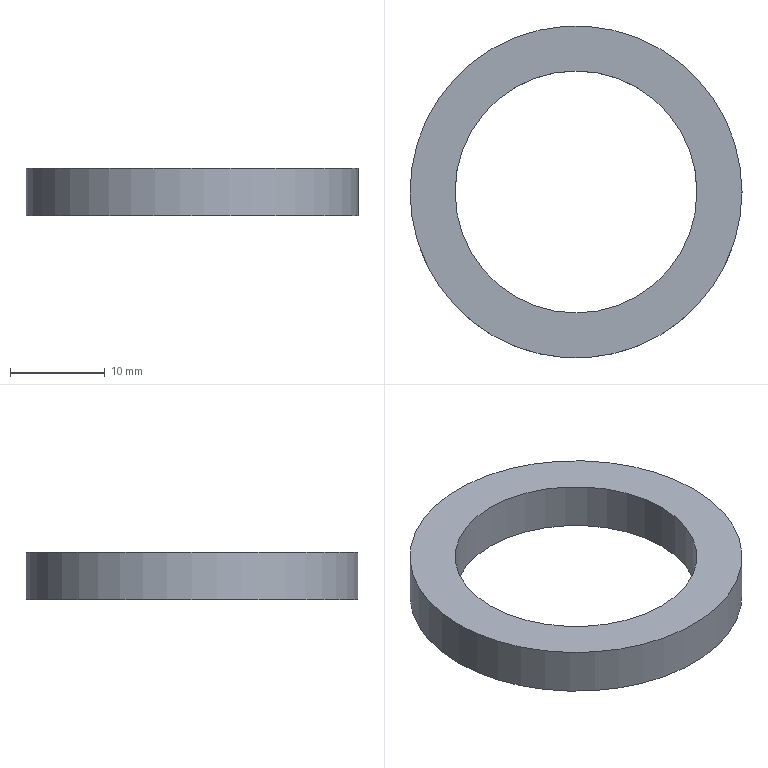Component | NX | SHAFT_SLEEVE_1 | 1 solid | 4 faces | box 35 x 35 x 5 mm | volume 2257 mm3 | cylinder 2 | plane 2 | commonest cylinder face diameters 35 x1 25.5 x1
STEP:
#1=CARTESIAN_POINT('',(0.,0.,0.));
#2=DIRECTION('',(0.,0.,1.));
#3=DIRECTION('',(1.,0.,0.));
#4=AXIS2_PLACEMENT_3D('',#1,#2,#3);
#5=CARTESIAN_POINT('',(-406.675,308.181,-720.));
#6=VERTEX_POINT('',#5);
#7=CARTESIAN_POINT('',(-424.175,308.181,-720.));
#8=DIRECTION('',(0.,0.,1.));
#9=DIRECTION('',(1.,0.,0.));
#10=AXIS2_PLACEMENT_3D('',#7,#8,#9);
#11=CIRCLE('',#10,17.5);
#12=CARTESIAN_POINT('',(-424.175,308.181,-720.));
#13=DIRECTION('',(0.,0.,-1.));
#14=DIRECTION('',(-1.,0.,0.));
#15=AXIS2_PLACEMENT_3D('',#12,#13,#14);
#16=CYLINDRICAL_SURFACE('',#15,17.5);
#17=CARTESIAN_POINT('',(9.425,0.));
#18=DIRECTION('',(-1.,0.));
#19=VECTOR('',#18,1.);
#20=LINE('',#17,#19);
#21=(GEOMETRIC_REPRESENTATION_CONTEXT(2)PARAMETRIC_REPRESENTATION_CONTEXT()REPRESENTATION_CONTEXT('',''));
#22=DEFINITIONAL_REPRESENTATION('',(#20),#21);
#23=PCURVE('',#16,#22);
#24=CARTESIAN_POINT('',(-424.175,308.181,-720.));
#25=DIRECTION('',(0.,0.,1.));
#26=DIRECTION('',(1.,0.,0.));
#27=AXIS2_PLACEMENT_3D('',#24,#25,#26);
#28=PLANE('',#27);
#29=CARTESIAN_POINT('',(0.,0.));
#30=DIRECTION('',(1.,0.));
#31=AXIS2_PLACEMENT_2D('',#29,#30);
#32=CIRCLE('',#31,17.5);
#33=(GEOMETRIC_REPRESENTATION_CONTEXT(2)PARAMETRIC_REPRESENTATION_CONTEXT()REPRESENTATION_CONTEXT('',''));
#34=DEFINITIONAL_REPRESENTATION('',(#32),#33);
#35=PCURVE('',#28,#34);
#36=SURFACE_CURVE('',#11,(#23,#35),.PCURVE_S1.);
#37=EDGE_CURVE('',#6,#6,#36,.T.);
#38=ORIENTED_EDGE('',*,*,#37,.F.);
#39=CARTESIAN_POINT('',(-406.675,308.181,-725.));
#40=VERTEX_POINT('',#39);
#41=CARTESIAN_POINT('',(-406.675,308.181,-720.));
#42=CARTESIAN_POINT('',(-406.675,308.181,-725.));
#43=B_SPLINE_CURVE_WITH_KNOTS('',1,(#41,#42),.UNSPECIFIED.,.F.,.F.,(2,2),(0.,5.),.PIECEWISE_BEZIER_KNOTS.);
#44=CARTESIAN_POINT('',(9.425,0.));
#45=DIRECTION('',(0.,1.));
#46=VECTOR('',#45,1.);
#47=LINE('',#44,#46);
#48=(GEOMETRIC_REPRESENTATION_CONTEXT(2)PARAMETRIC_REPRESENTATION_CONTEXT()REPRESENTATION_CONTEXT('',''));
#49=DEFINITIONAL_REPRESENTATION('',(#47),#48);
#50=PCURVE('',#16,#49);
#51=CARTESIAN_POINT('',(3.142,0.));
#52=DIRECTION('',(0.,1.));
#53=VECTOR('',#52,1.);
#54=LINE('',#51,#53);
#55=(GEOMETRIC_REPRESENTATION_CONTEXT(2)PARAMETRIC_REPRESENTATION_CONTEXT()REPRESENTATION_CONTEXT('',''));
#56=DEFINITIONAL_REPRESENTATION('',(#54),#55);
#57=PCURVE('',#16,#56);
#58=SEAM_CURVE('',#43,(#50,#57),.PCURVE_S1.);
#59=EDGE_CURVE('',#6,#40,#58,.T.);
#60=ORIENTED_EDGE('',*,*,#59,.T.);
#61=CARTESIAN_POINT('',(-424.175,308.181,-725.));
#62=DIRECTION('',(0.,0.,1.));
#63=DIRECTION('',(1.,0.,0.));
#64=AXIS2_PLACEMENT_3D('',#61,#62,#63);
#65=CIRCLE('',#64,17.5);
#66=CARTESIAN_POINT('',(9.425,5.));
#67=DIRECTION('',(-1.,0.));
#68=VECTOR('',#67,1.);
#69=LINE('',#66,#68);
#70=(GEOMETRIC_REPRESENTATION_CONTEXT(2)PARAMETRIC_REPRESENTATION_CONTEXT()REPRESENTATION_CONTEXT('',''));
#71=DEFINITIONAL_REPRESENTATION('',(#69),#70);
#72=PCURVE('',#16,#71);
#73=CARTESIAN_POINT('',(-424.175,308.181,-725.));
#74=DIRECTION('',(0.,0.,1.));
#75=DIRECTION('',(1.,0.,0.));
#76=AXIS2_PLACEMENT_3D('',#73,#74,#75);
#77=PLANE('',#76);
#78=CARTESIAN_POINT('',(0.,0.));
#79=DIRECTION('',(1.,0.));
#80=AXIS2_PLACEMENT_2D('',#78,#79);
#81=CIRCLE('',#80,17.5);
#82=(GEOMETRIC_REPRESENTATION_CONTEXT(2)PARAMETRIC_REPRESENTATION_CONTEXT()REPRESENTATION_CONTEXT('',''));
#83=DEFINITIONAL_REPRESENTATION('',(#81),#82);
#84=PCURVE('',#77,#83);
#85=SURFACE_CURVE('',#65,(#72,#84),.PCURVE_S1.);
#86=EDGE_CURVE('',#40,#40,#85,.T.);
#87=ORIENTED_EDGE('',*,*,#86,.T.);
#88=ORIENTED_EDGE('',*,*,#59,.F.);
#89=EDGE_LOOP('',(#38,#60,#87,#88));
#90=FACE_BOUND('',#89,.T.);
#91=ADVANCED_FACE('',(#90),#16,.T.);
#92=CARTESIAN_POINT('',(-411.425,308.181,-720.));
#93=VERTEX_POINT('',#92);
#94=CARTESIAN_POINT('',(-424.175,308.181,-720.));
#95=DIRECTION('',(0.,0.,1.));
#96=DIRECTION('',(1.,0.,0.));
#97=AXIS2_PLACEMENT_3D('',#94,#95,#96);
#98=CIRCLE('',#97,12.75);
#99=CARTESIAN_POINT('',(-424.175,308.181,-720.));
#100=DIRECTION('',(0.,0.,-1.));
#101=DIRECTION('',(-1.,0.,0.));
#102=AXIS2_PLACEMENT_3D('',#99,#100,#101);
#103=CYLINDRICAL_SURFACE('',#102,12.75);
#104=CARTESIAN_POINT('',(9.425,0.));
#105=DIRECTION('',(-1.,0.));
#106=VECTOR('',#105,1.);
#107=LINE('',#104,#106);
#108=(GEOMETRIC_REPRESENTATION_CONTEXT(2)PARAMETRIC_REPRESENTATION_CONTEXT()REPRESENTATION_CONTEXT('',''));
#109=DEFINITIONAL_REPRESENTATION('',(#107),#108);
#110=PCURVE('',#103,#109);
#111=CARTESIAN_POINT('',(0.,0.));
#112=DIRECTION('',(1.,0.));
#113=AXIS2_PLACEMENT_2D('',#111,#112);
#114=CIRCLE('',#113,12.75);
#115=(GEOMETRIC_REPRESENTATION_CONTEXT(2)PARAMETRIC_REPRESENTATION_CONTEXT()REPRESENTATION_CONTEXT('',''));
#116=DEFINITIONAL_REPRESENTATION('',(#114),#115);
#117=PCURVE('',#28,#116);
#118=SURFACE_CURVE('',#98,(#110,#117),.PCURVE_S1.);
#119=EDGE_CURVE('',#93,#93,#118,.T.);
#120=ORIENTED_EDGE('',*,*,#119,.F.);
#121=CARTESIAN_POINT('',(-411.425,308.181,-725.));
#122=VERTEX_POINT('',#121);
#123=CARTESIAN_POINT('',(-411.425,308.181,-720.));
#124=CARTESIAN_POINT('',(-411.425,308.181,-725.));
#125=B_SPLINE_CURVE_WITH_KNOTS('',1,(#123,#124),.UNSPECIFIED.,.F.,.F.,(2,2),(0.,5.),.PIECEWISE_BEZIER_KNOTS.);
#126=CARTESIAN_POINT('',(9.425,0.));
#127=DIRECTION('',(0.,1.));
#128=VECTOR('',#127,1.);
#129=LINE('',#126,#128);
#130=(GEOMETRIC_REPRESENTATION_CONTEXT(2)PARAMETRIC_REPRESENTATION_CONTEXT()REPRESENTATION_CONTEXT('',''));
#131=DEFINITIONAL_REPRESENTATION('',(#129),#130);
#132=PCURVE('',#103,#131);
#133=CARTESIAN_POINT('',(3.142,0.));
#134=DIRECTION('',(0.,1.));
#135=VECTOR('',#134,1.);
#136=LINE('',#133,#135);
#137=(GEOMETRIC_REPRESENTATION_CONTEXT(2)PARAMETRIC_REPRESENTATION_CONTEXT()REPRESENTATION_CONTEXT('',''));
#138=DEFINITIONAL_REPRESENTATION('',(#136),#137);
#139=PCURVE('',#103,#138);
#140=SEAM_CURVE('',#125,(#132,#139),.PCURVE_S1.);
#141=EDGE_CURVE('',#93,#122,#140,.T.);
#142=ORIENTED_EDGE('',*,*,#141,.T.);
#143=CARTESIAN_POINT('',(-424.175,308.181,-725.));
#144=DIRECTION('',(0.,0.,1.));
#145=DIRECTION('',(1.,0.,0.));
#146=AXIS2_PLACEMENT_3D('',#143,#144,#145);
#147=CIRCLE('',#146,12.75);
#148=CARTESIAN_POINT('',(9.425,5.));
#149=DIRECTION('',(-1.,0.));
#150=VECTOR('',#149,1.);
#151=LINE('',#148,#150);
#152=(GEOMETRIC_REPRESENTATION_CONTEXT(2)PARAMETRIC_REPRESENTATION_CONTEXT()REPRESENTATION_CONTEXT('',''));
#153=DEFINITIONAL_REPRESENTATION('',(#151),#152);
#154=PCURVE('',#103,#153);
#155=CARTESIAN_POINT('',(0.,0.));
#156=DIRECTION('',(1.,0.));
#157=AXIS2_PLACEMENT_2D('',#155,#156);
#158=CIRCLE('',#157,12.75);
#159=(GEOMETRIC_REPRESENTATION_CONTEXT(2)PARAMETRIC_REPRESENTATION_CONTEXT()REPRESENTATION_CONTEXT('',''));
#160=DEFINITIONAL_REPRESENTATION('',(#158),#159);
#161=PCURVE('',#77,#160);
#162=SURFACE_CURVE('',#147,(#154,#161),.PCURVE_S1.);
#163=EDGE_CURVE('',#122,#122,#162,.T.);
#164=ORIENTED_EDGE('',*,*,#163,.T.);
#165=ORIENTED_EDGE('',*,*,#141,.F.);
#166=EDGE_LOOP('',(#120,#142,#164,#165));
#167=FACE_BOUND('',#166,.F.);
#168=ADVANCED_FACE('',(#167),#103,.F.);
#169=ORIENTED_EDGE('',*,*,#37,.T.);
#170=EDGE_LOOP('',(#169));
#171=FACE_BOUND('',#170,.T.);
#172=ORIENTED_EDGE('',*,*,#119,.F.);
#173=EDGE_LOOP('',(#172));
#174=FACE_BOUND('',#173,.T.);
#175=ADVANCED_FACE('',(#171,#174),#28,.T.);
#176=ORIENTED_EDGE('',*,*,#86,.F.);
#177=EDGE_LOOP('',(#176));
#178=FACE_BOUND('',#177,.T.);
#179=ORIENTED_EDGE('',*,*,#163,.T.);
#180=EDGE_LOOP('',(#179));
#181=FACE_BOUND('',#180,.T.);
#182=ADVANCED_FACE('',(#178,#181),#77,.F.);
#183=CLOSED_SHELL('',(#91,#168,#175,#182));
#184=MANIFOLD_SOLID_BREP('',#183);
#185=(LENGTH_UNIT()NAMED_UNIT(*)SI_UNIT(.MILLI.,.METRE.));
#186=UNCERTAINTY_MEASURE_WITH_UNIT(LENGTH_MEASURE(0.00001),#185,'','');
#187=(NAMED_UNIT(*)PLANE_ANGLE_UNIT()SI_UNIT($,.RADIAN.));
#188=(NAMED_UNIT(*)SI_UNIT($,.STERADIAN.)SOLID_ANGLE_UNIT());
#189=(GEOMETRIC_REPRESENTATION_CONTEXT(3)GLOBAL_UNCERTAINTY_ASSIGNED_CONTEXT((#186))GLOBAL_UNIT_ASSIGNED_CONTEXT((#185,#187,#188))REPRESENTATION_CONTEXT('',''));
#190=ADVANCED_BREP_SHAPE_REPRESENTATION('',(#4,#184),#189);